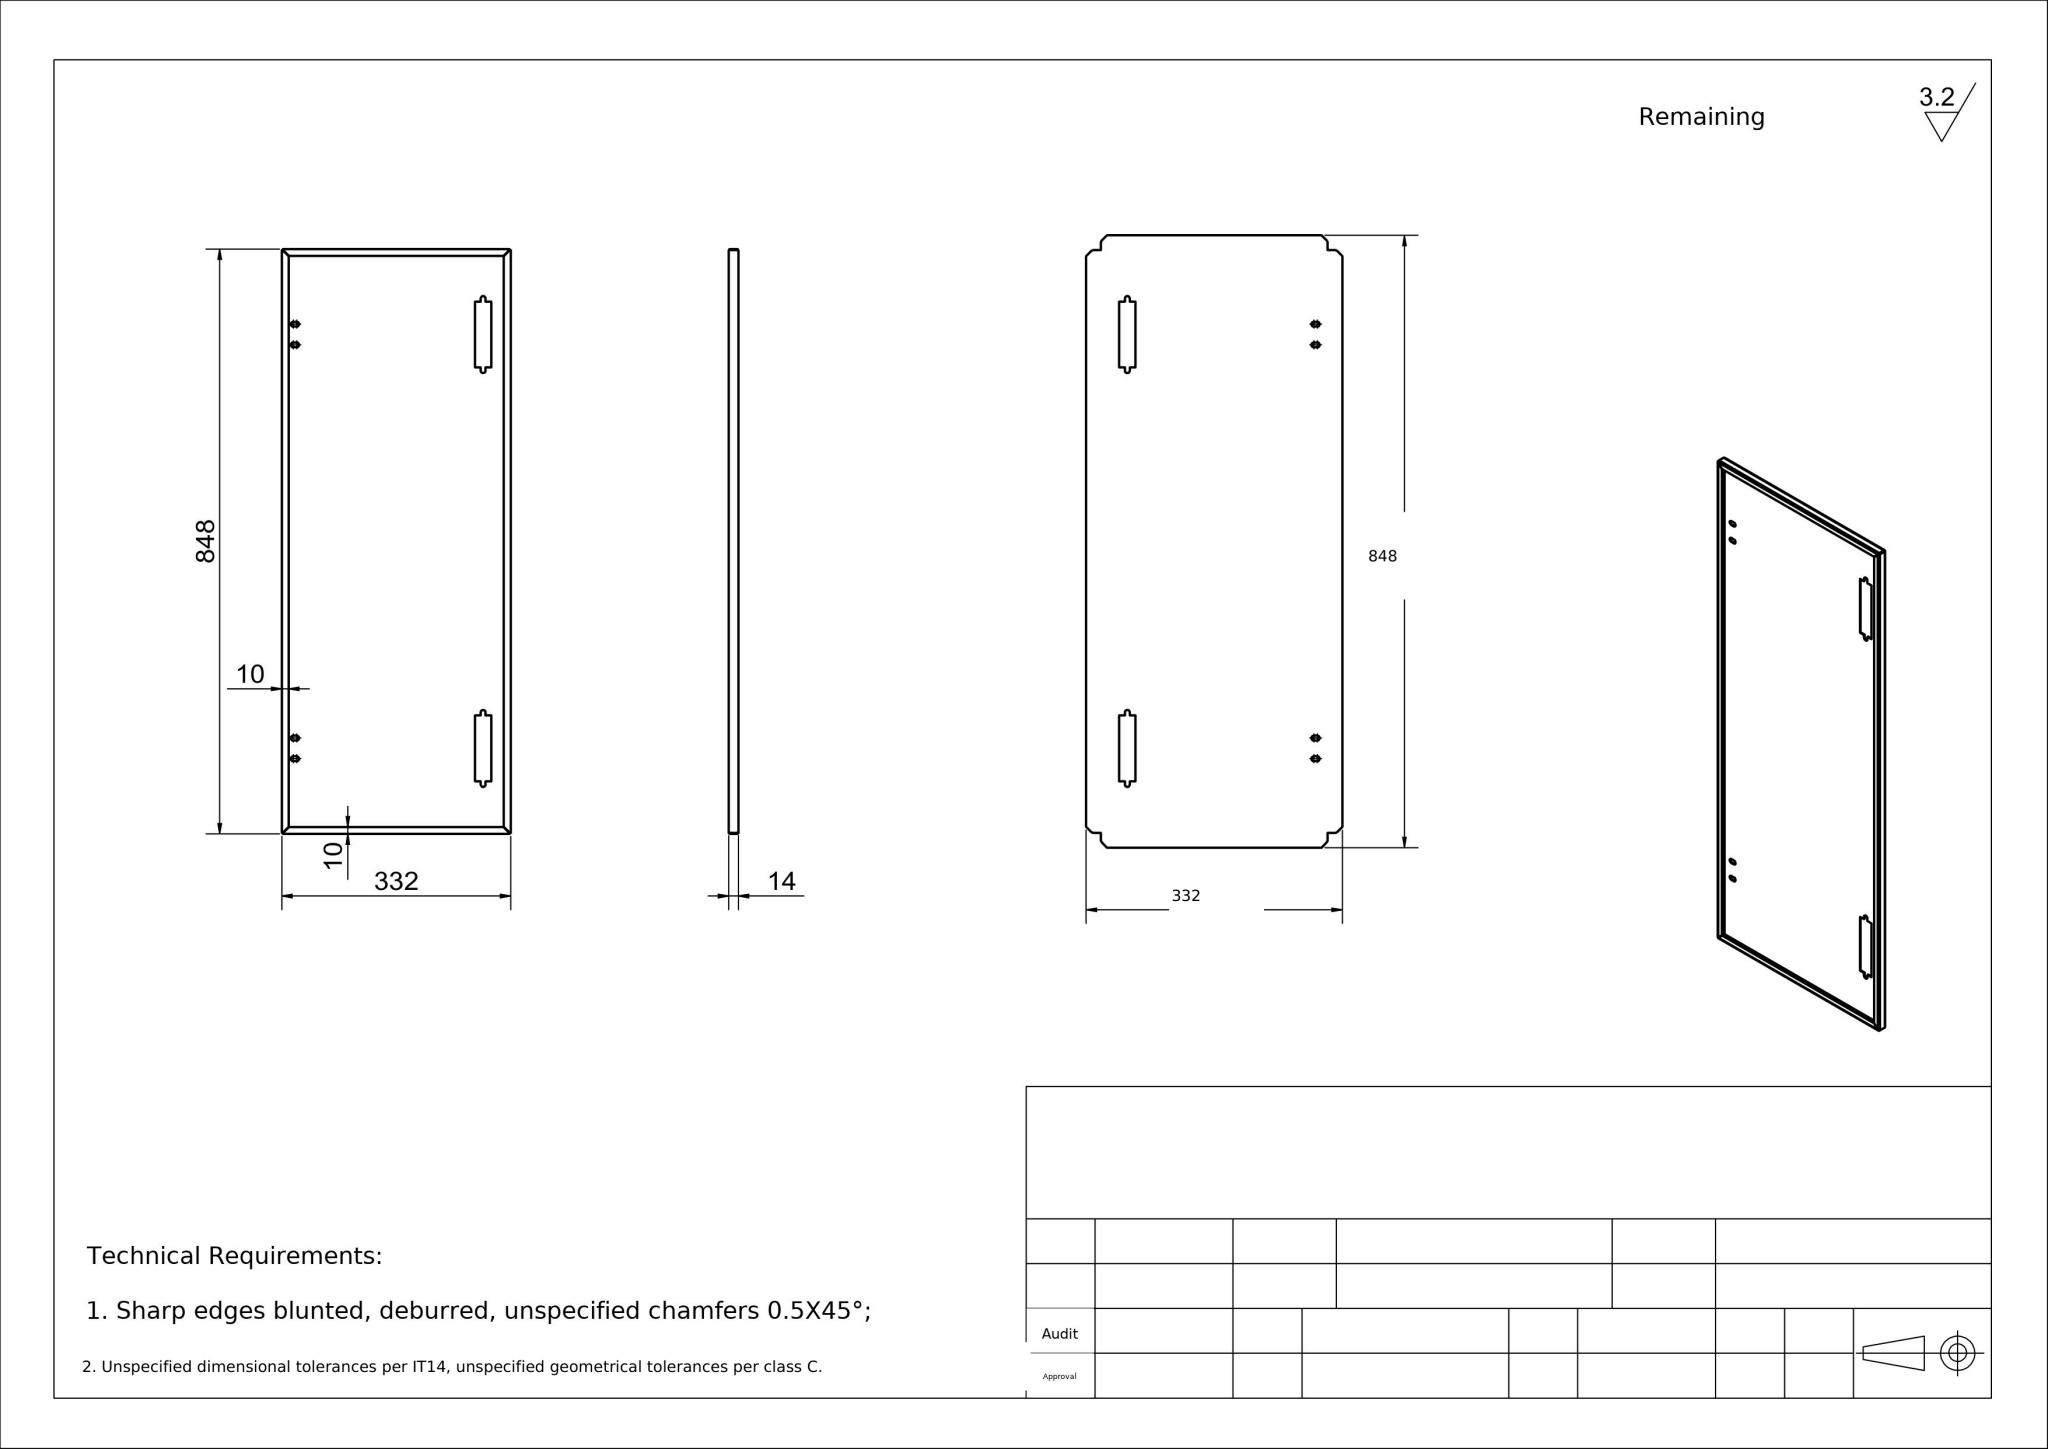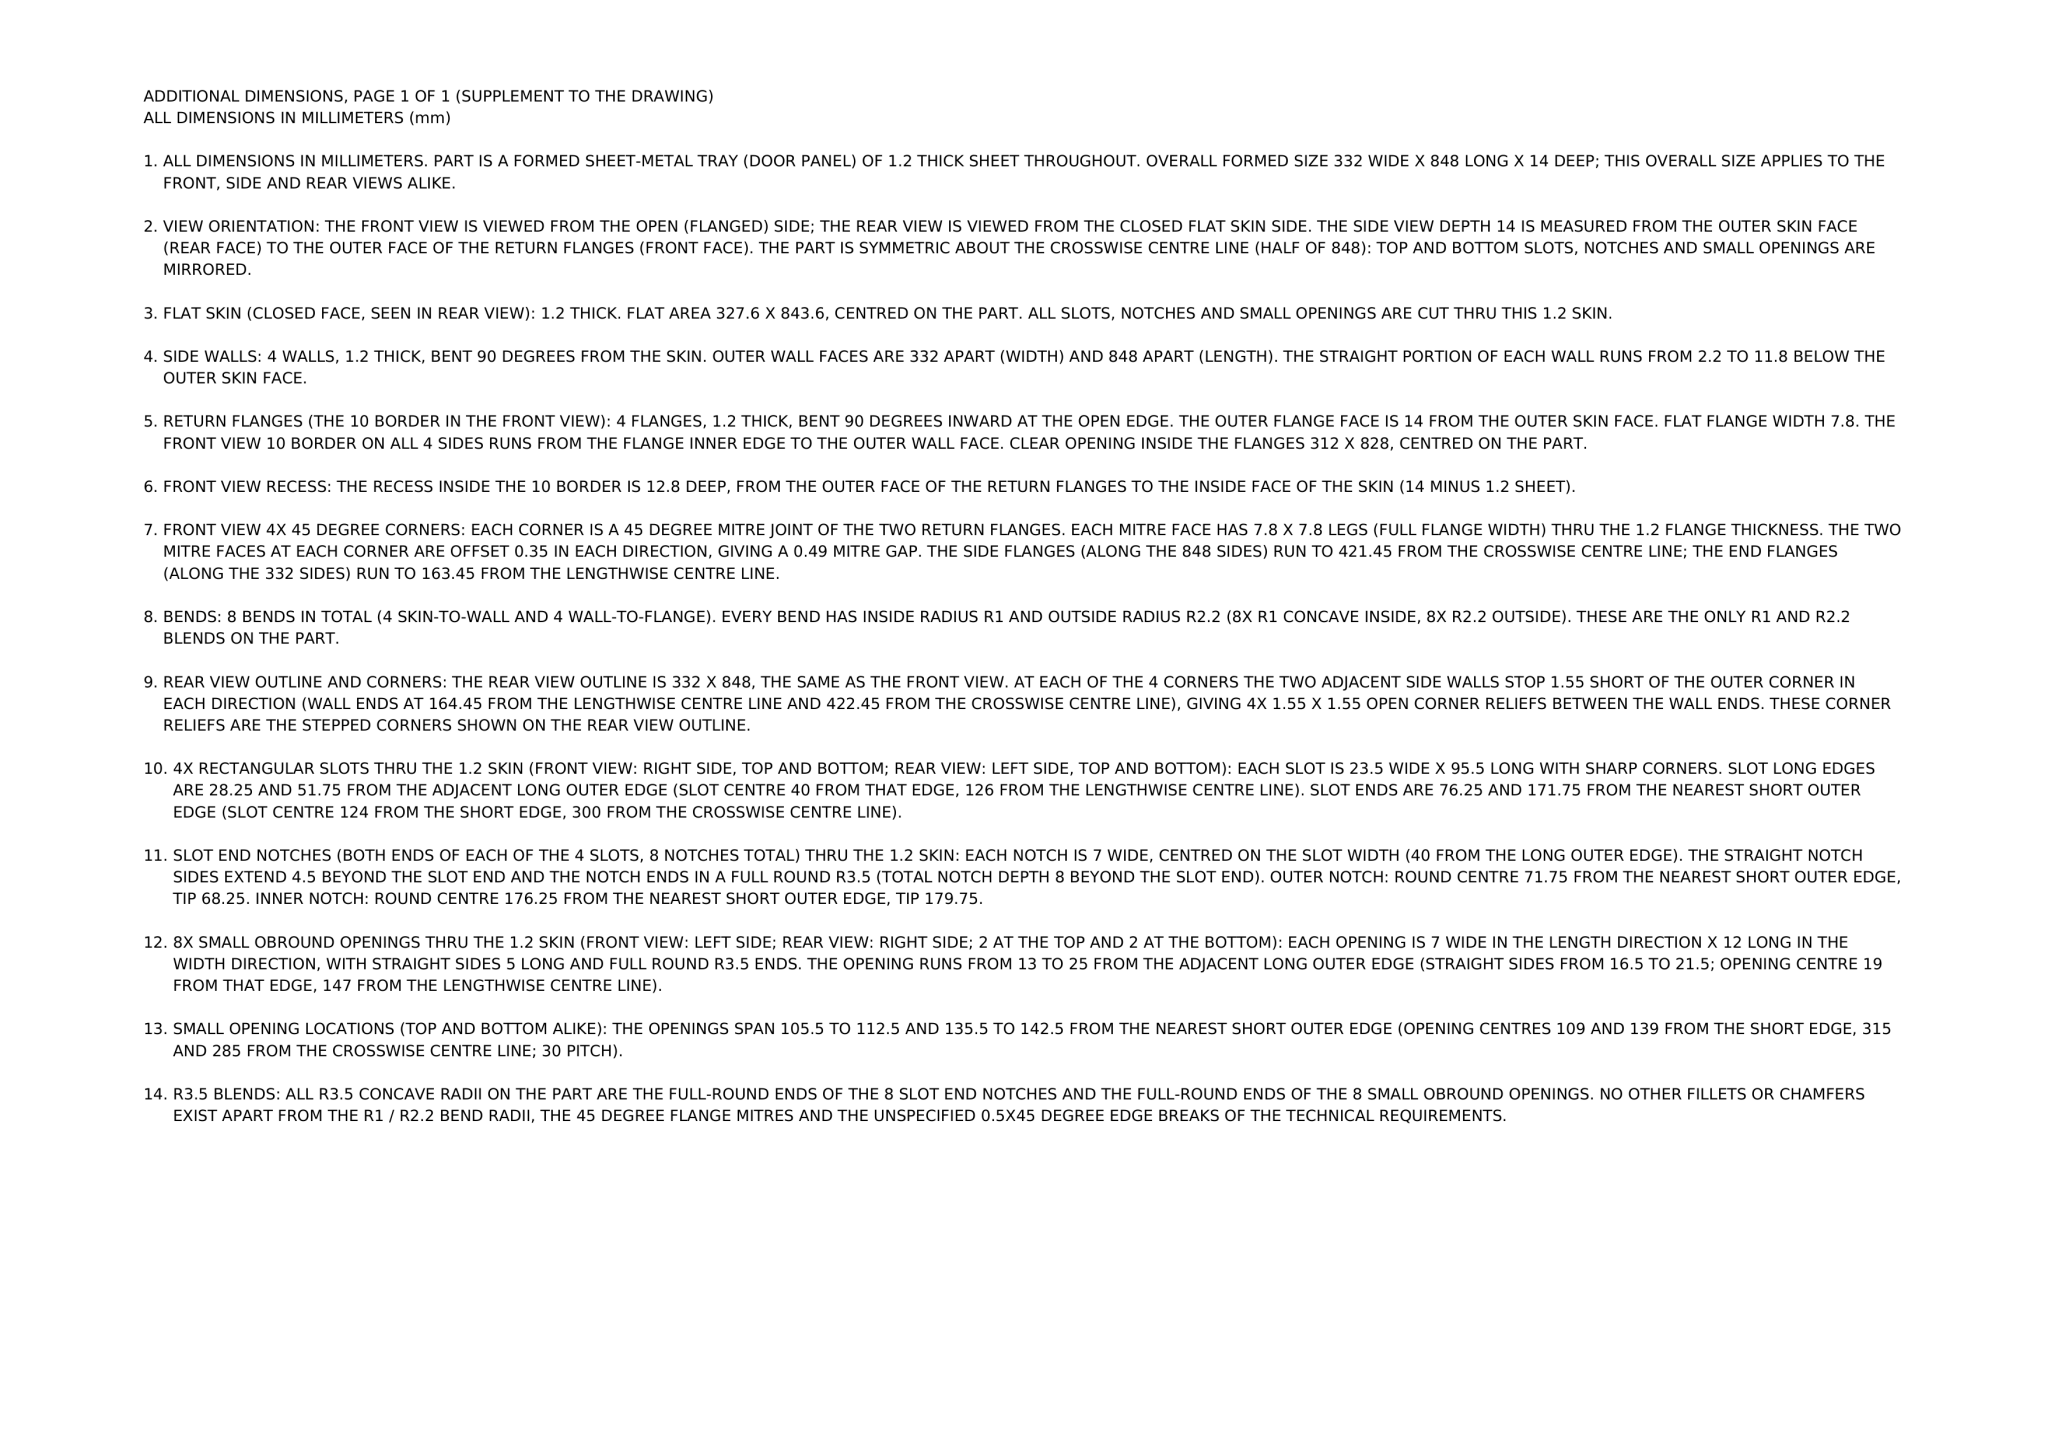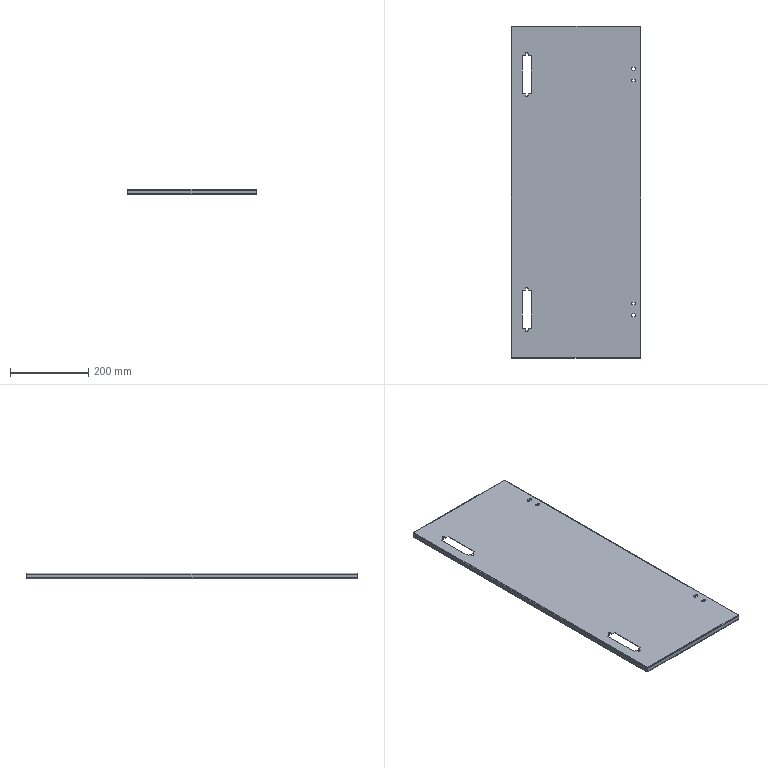Part | NX | mm | 1 solid | 114 faces | box 332 x 848 x 14 mm | volume 388444 mm3 | plane 66 | cylinder 32 | spline 16 | commonest cylinder face diameters 7 x16 4.4 x8 2 x8